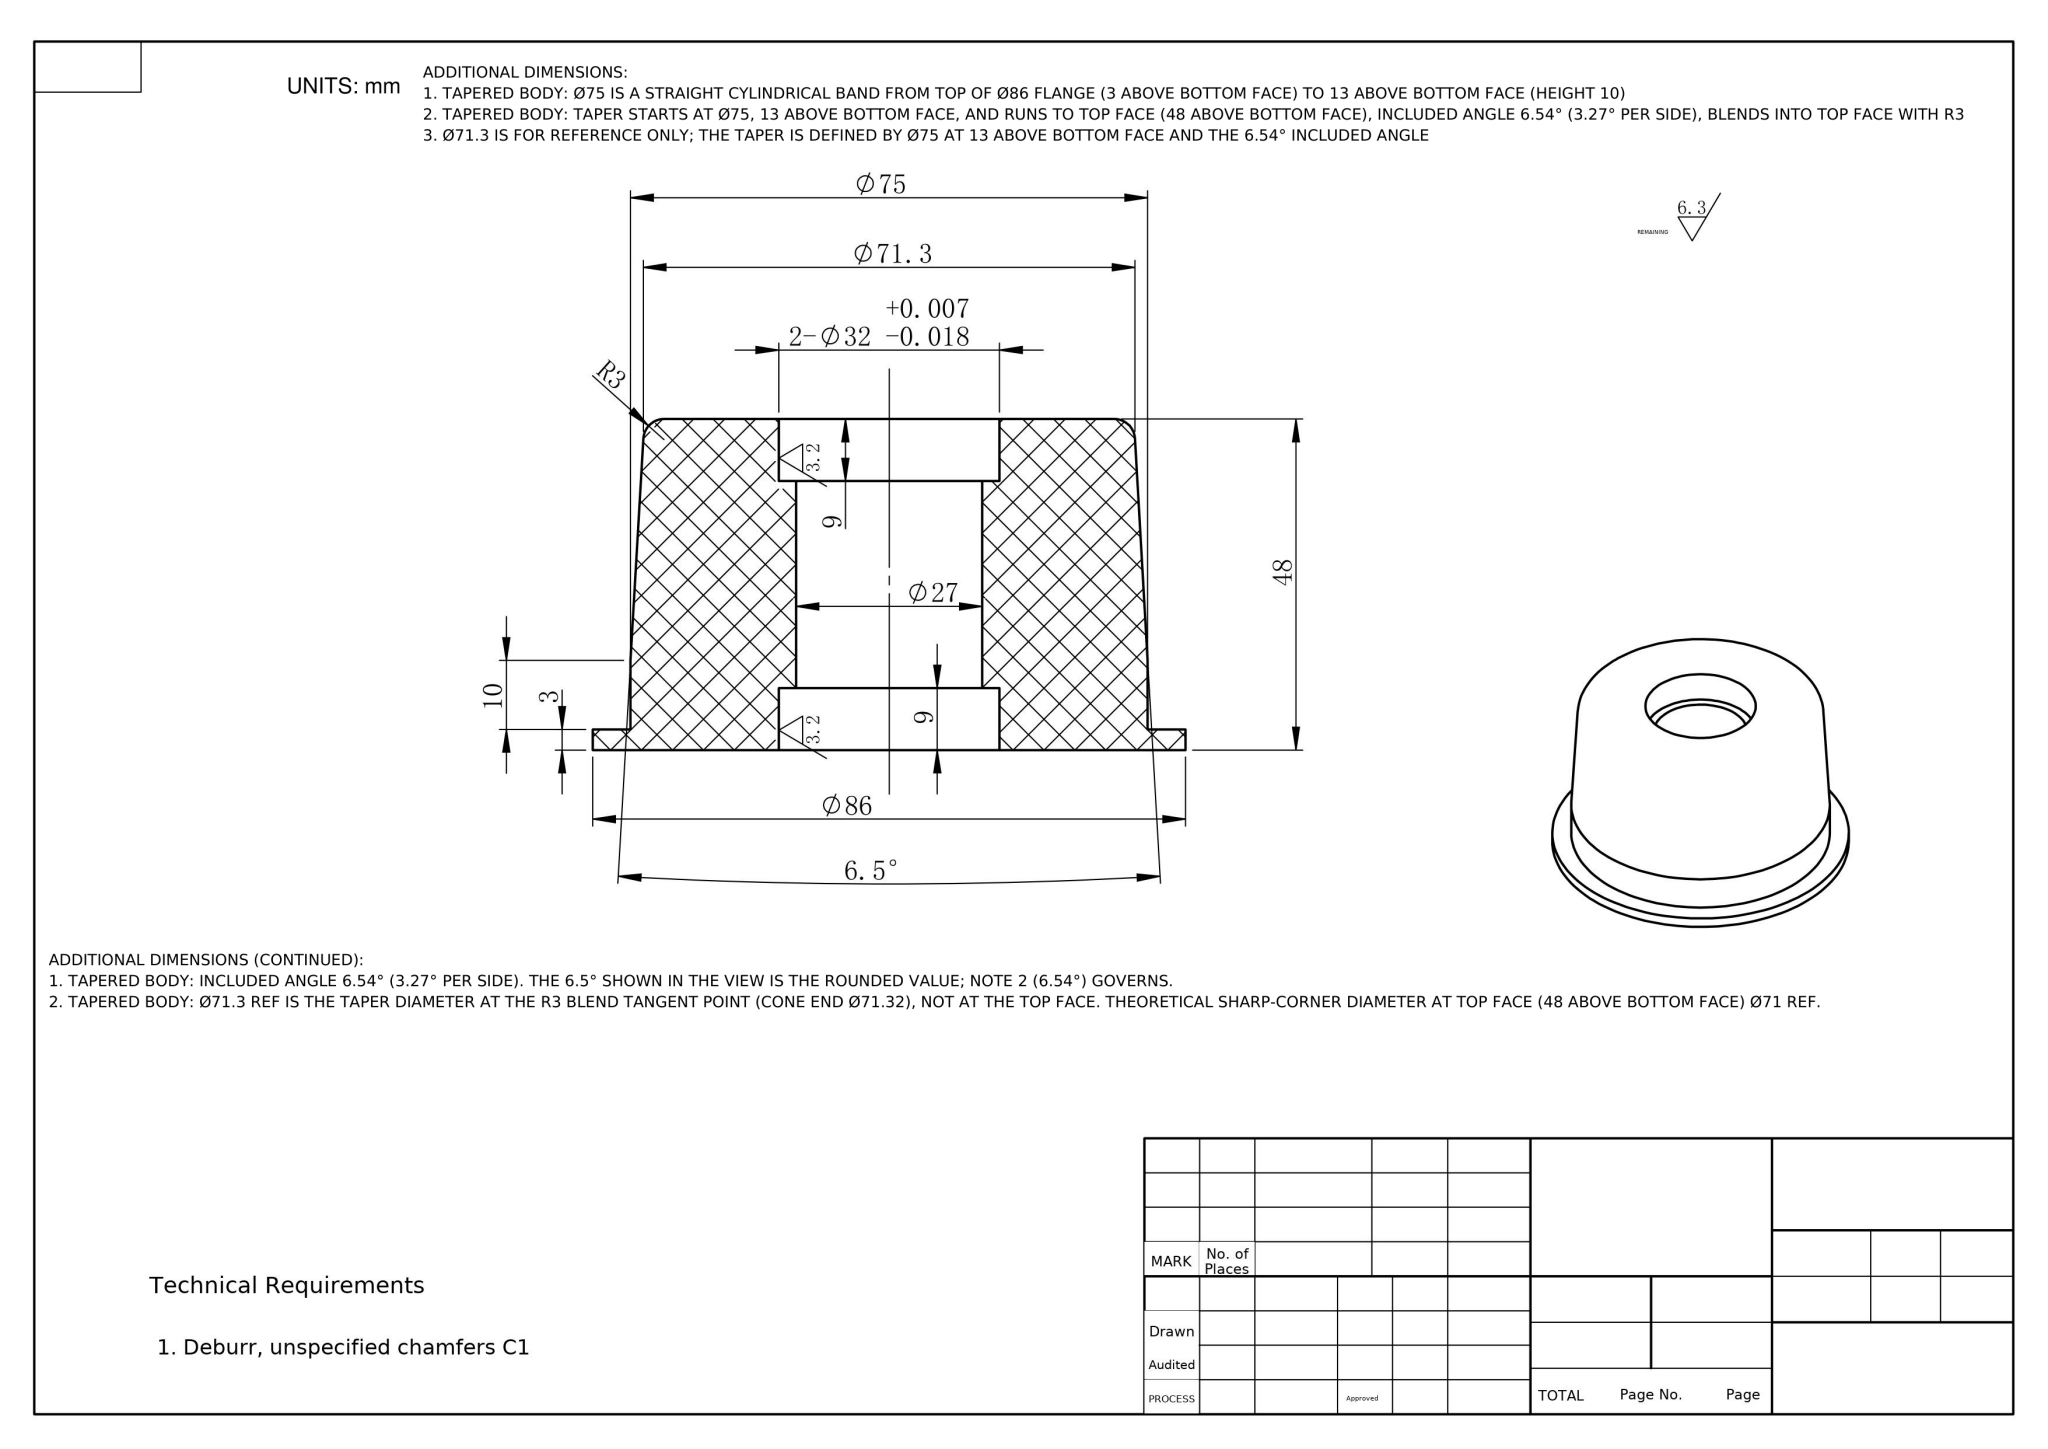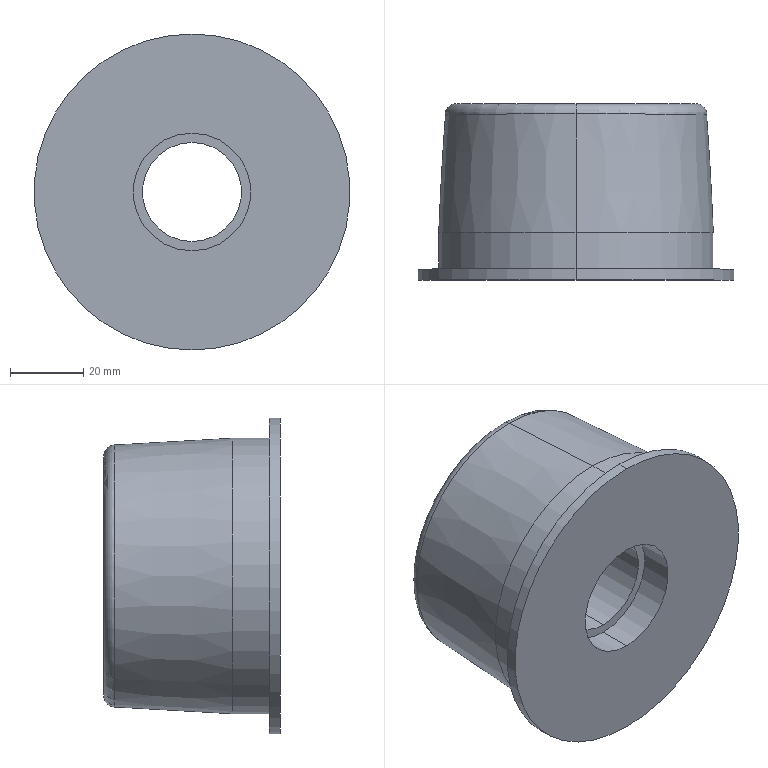Part | NX | mm | 1 solid | 19 faces | box 86 x 48 x 86 mm | volume 176107 mm3 | cylinder 10 | plane 5 | torus 2 | cone 2 | commonest cylinder face diameters 32 x4 75 x2 86 x2 27 x2
STEP:
#1=COLOUR_RGB('',0.9882,0.7373,0.5176);
#2=FILL_AREA_STYLE_COLOUR('',#1);
#3=FILL_AREA_STYLE('',(#2));
#4=SURFACE_STYLE_FILL_AREA(#3);
#5=SURFACE_SIDE_STYLE('',(#4));
#6=SURFACE_STYLE_USAGE(.BOTH.,#5);
#7=PRESENTATION_STYLE_ASSIGNMENT((#6));
#8=CARTESIAN_POINT('',(0.,13.,-37.5));
#9=VERTEX_POINT('',#8);
#10=CARTESIAN_POINT('',(0.,13.,37.5));
#11=VERTEX_POINT('',#10);
#12=CARTESIAN_POINT('',(0.,13.,0.));
#13=DIRECTION('',(0.,-1.,0.));
#14=DIRECTION('',(0.,0.,-1.));
#15=AXIS2_PLACEMENT_3D('',#12,#13,#14);
#16=CIRCLE('',#15,37.5);
#17=EDGE_CURVE('',#9,#11,#16,.T.);
#18=ORIENTED_EDGE('',*,*,#17,.T.);
#19=CARTESIAN_POINT('',(0.,3.,37.5));
#20=VERTEX_POINT('',#19);
#21=CARTESIAN_POINT('',(0.,-3.006,37.5));
#22=DIRECTION('',(0.,-1.,0.));
#23=VECTOR('',#22,1000.);
#24=LINE('',#21,#23);
#25=EDGE_CURVE('',#11,#20,#24,.T.);
#26=ORIENTED_EDGE('',*,*,#25,.T.);
#27=CARTESIAN_POINT('',(0.,3.,-37.5));
#28=VERTEX_POINT('',#27);
#29=CARTESIAN_POINT('',(0.,3.,0.));
#30=DIRECTION('',(0.,-1.,0.));
#31=DIRECTION('',(0.,0.,-1.));
#32=AXIS2_PLACEMENT_3D('',#29,#30,#31);
#33=CIRCLE('',#32,37.5);
#34=EDGE_CURVE('',#28,#20,#33,.T.);
#35=ORIENTED_EDGE('',*,*,#34,.F.);
#36=CARTESIAN_POINT('',(0.,-3.006,-37.5));
#37=DIRECTION('',(0.,-1.,0.));
#38=VECTOR('',#37,1000.);
#39=LINE('',#36,#38);
#40=EDGE_CURVE('',#9,#28,#39,.T.);
#41=ORIENTED_EDGE('',*,*,#40,.F.);
#42=EDGE_LOOP('',(#18,#26,#35,#41));
#43=FACE_OUTER_BOUND('',#42,.T.);
#44=CARTESIAN_POINT('',(0.,-3.006,0.));
#45=DIRECTION('',(0.,-1.,0.));
#46=DIRECTION('',(0.,0.,-1.));
#47=AXIS2_PLACEMENT_3D('',#44,#45,#46);
#48=CYLINDRICAL_SURFACE('',#47,37.5);
#49=ADVANCED_FACE('',(#43),#48,.T.);
#50=CARTESIAN_POINT('',(0.,3.,-43.));
#51=VERTEX_POINT('',#50);
#52=CARTESIAN_POINT('',(0.,3.,43.));
#53=VERTEX_POINT('',#52);
#54=CARTESIAN_POINT('',(0.,3.,0.));
#55=DIRECTION('',(0.,-1.,0.));
#56=DIRECTION('',(0.,0.,-1.));
#57=AXIS2_PLACEMENT_3D('',#54,#55,#56);
#58=CIRCLE('',#57,43.);
#59=EDGE_CURVE('',#51,#53,#58,.T.);
#60=ORIENTED_EDGE('',*,*,#59,.T.);
#61=CARTESIAN_POINT('',(0.,0.,43.));
#62=VERTEX_POINT('',#61);
#63=CARTESIAN_POINT('',(0.,-3.006,43.));
#64=DIRECTION('',(0.,-1.,0.));
#65=VECTOR('',#64,1000.);
#66=LINE('',#63,#65);
#67=EDGE_CURVE('',#53,#62,#66,.T.);
#68=ORIENTED_EDGE('',*,*,#67,.T.);
#69=CARTESIAN_POINT('',(0.,0.,-43.));
#70=VERTEX_POINT('',#69);
#71=CARTESIAN_POINT('',(0.,0.,0.));
#72=DIRECTION('',(0.,-1.,0.));
#73=DIRECTION('',(0.,0.,-1.));
#74=AXIS2_PLACEMENT_3D('',#71,#72,#73);
#75=CIRCLE('',#74,43.);
#76=EDGE_CURVE('',#70,#62,#75,.T.);
#77=ORIENTED_EDGE('',*,*,#76,.F.);
#78=CARTESIAN_POINT('',(0.,-3.006,-43.));
#79=DIRECTION('',(0.,-1.,0.));
#80=VECTOR('',#79,1000.);
#81=LINE('',#78,#80);
#82=EDGE_CURVE('',#51,#70,#81,.T.);
#83=ORIENTED_EDGE('',*,*,#82,.F.);
#84=EDGE_LOOP('',(#60,#68,#77,#83));
#85=FACE_OUTER_BOUND('',#84,.T.);
#86=CARTESIAN_POINT('',(0.,-3.006,0.));
#87=DIRECTION('',(0.,-1.,0.));
#88=DIRECTION('',(0.,0.,-1.));
#89=AXIS2_PLACEMENT_3D('',#86,#87,#88);
#90=CYLINDRICAL_SURFACE('',#89,43.);
#91=ADVANCED_FACE('',(#85),#90,.T.);
#92=CARTESIAN_POINT('',(0.,9.,16.));
#93=VERTEX_POINT('',#92);
#94=CARTESIAN_POINT('',(0.,9.,-16.));
#95=VERTEX_POINT('',#94);
#96=CARTESIAN_POINT('',(0.,9.,0.));
#97=DIRECTION('',(0.,-1.,0.));
#98=DIRECTION('',(0.,0.,-1.));
#99=AXIS2_PLACEMENT_3D('',#96,#97,#98);
#100=CIRCLE('',#99,16.);
#101=EDGE_CURVE('',#93,#95,#100,.T.);
#102=ORIENTED_EDGE('',*,*,#101,.F.);
#103=CARTESIAN_POINT('',(0.,0.,16.));
#104=VERTEX_POINT('',#103);
#105=CARTESIAN_POINT('',(0.,-3.006,16.));
#106=DIRECTION('',(0.,-1.,0.));
#107=VECTOR('',#106,1000.);
#108=LINE('',#105,#107);
#109=EDGE_CURVE('',#93,#104,#108,.T.);
#110=ORIENTED_EDGE('',*,*,#109,.T.);
#111=CARTESIAN_POINT('',(0.,0.,-16.));
#112=VERTEX_POINT('',#111);
#113=CARTESIAN_POINT('',(0.,0.,0.));
#114=DIRECTION('',(0.,-1.,0.));
#115=DIRECTION('',(0.,0.,-1.));
#116=AXIS2_PLACEMENT_3D('',#113,#114,#115);
#117=CIRCLE('',#116,16.);
#118=EDGE_CURVE('',#104,#112,#117,.T.);
#119=ORIENTED_EDGE('',*,*,#118,.T.);
#120=CARTESIAN_POINT('',(0.,-3.006,-16.));
#121=DIRECTION('',(0.,-1.,0.));
#122=VECTOR('',#121,1000.);
#123=LINE('',#120,#122);
#124=EDGE_CURVE('',#95,#112,#123,.T.);
#125=ORIENTED_EDGE('',*,*,#124,.F.);
#126=EDGE_LOOP('',(#102,#110,#119,#125));
#127=FACE_OUTER_BOUND('',#126,.T.);
#128=CARTESIAN_POINT('',(0.,-3.006,0.));
#129=DIRECTION('',(0.,-1.,0.));
#130=DIRECTION('',(0.,0.,-1.));
#131=AXIS2_PLACEMENT_3D('',#128,#129,#130);
#132=CYLINDRICAL_SURFACE('',#131,16.);
#133=ADVANCED_FACE('',(#127),#132,.F.);
#134=CARTESIAN_POINT('',(0.,39.,13.5));
#135=VERTEX_POINT('',#134);
#136=CARTESIAN_POINT('',(0.,39.,-13.5));
#137=VERTEX_POINT('',#136);
#138=CARTESIAN_POINT('',(0.,39.,0.));
#139=DIRECTION('',(0.,-1.,0.));
#140=DIRECTION('',(0.,0.,-1.));
#141=AXIS2_PLACEMENT_3D('',#138,#139,#140);
#142=CIRCLE('',#141,13.5);
#143=EDGE_CURVE('',#135,#137,#142,.T.);
#144=ORIENTED_EDGE('',*,*,#143,.F.);
#145=CARTESIAN_POINT('',(0.,9.,13.5));
#146=VERTEX_POINT('',#145);
#147=CARTESIAN_POINT('',(0.,-3.006,13.5));
#148=DIRECTION('',(0.,-1.,0.));
#149=VECTOR('',#148,1000.);
#150=LINE('',#147,#149);
#151=EDGE_CURVE('',#135,#146,#150,.T.);
#152=ORIENTED_EDGE('',*,*,#151,.T.);
#153=CARTESIAN_POINT('',(0.,9.,-13.5));
#154=VERTEX_POINT('',#153);
#155=CARTESIAN_POINT('',(0.,9.,0.));
#156=DIRECTION('',(0.,-1.,0.));
#157=DIRECTION('',(0.,0.,-1.));
#158=AXIS2_PLACEMENT_3D('',#155,#156,#157);
#159=CIRCLE('',#158,13.5);
#160=EDGE_CURVE('',#146,#154,#159,.T.);
#161=ORIENTED_EDGE('',*,*,#160,.T.);
#162=CARTESIAN_POINT('',(0.,-3.006,-13.5));
#163=DIRECTION('',(0.,-1.,0.));
#164=VECTOR('',#163,1000.);
#165=LINE('',#162,#164);
#166=EDGE_CURVE('',#137,#154,#165,.T.);
#167=ORIENTED_EDGE('',*,*,#166,.F.);
#168=EDGE_LOOP('',(#144,#152,#161,#167));
#169=FACE_OUTER_BOUND('',#168,.T.);
#170=CARTESIAN_POINT('',(0.,-3.006,0.));
#171=DIRECTION('',(0.,-1.,0.));
#172=DIRECTION('',(0.,0.,-1.));
#173=AXIS2_PLACEMENT_3D('',#170,#171,#172);
#174=CYLINDRICAL_SURFACE('',#173,13.5);
#175=ADVANCED_FACE('',(#169),#174,.F.);
#176=CARTESIAN_POINT('',(0.,48.,16.));
#177=VERTEX_POINT('',#176);
#178=CARTESIAN_POINT('',(0.,48.,-16.));
#179=VERTEX_POINT('',#178);
#180=CARTESIAN_POINT('',(0.,48.,0.));
#181=DIRECTION('',(0.,-1.,0.));
#182=DIRECTION('',(0.,0.,-1.));
#183=AXIS2_PLACEMENT_3D('',#180,#181,#182);
#184=CIRCLE('',#183,16.);
#185=EDGE_CURVE('',#177,#179,#184,.T.);
#186=ORIENTED_EDGE('',*,*,#185,.F.);
#187=CARTESIAN_POINT('',(0.,39.,16.));
#188=VERTEX_POINT('',#187);
#189=CARTESIAN_POINT('',(0.,-3.006,16.));
#190=DIRECTION('',(0.,-1.,0.));
#191=VECTOR('',#190,1000.);
#192=LINE('',#189,#191);
#193=EDGE_CURVE('',#177,#188,#192,.T.);
#194=ORIENTED_EDGE('',*,*,#193,.T.);
#195=CARTESIAN_POINT('',(0.,39.,-16.));
#196=VERTEX_POINT('',#195);
#197=CARTESIAN_POINT('',(0.,39.,0.));
#198=DIRECTION('',(0.,-1.,0.));
#199=DIRECTION('',(0.,0.,-1.));
#200=AXIS2_PLACEMENT_3D('',#197,#198,#199);
#201=CIRCLE('',#200,16.);
#202=EDGE_CURVE('',#188,#196,#201,.T.);
#203=ORIENTED_EDGE('',*,*,#202,.T.);
#204=CARTESIAN_POINT('',(0.,-3.006,-16.));
#205=DIRECTION('',(0.,-1.,0.));
#206=VECTOR('',#205,1000.);
#207=LINE('',#204,#206);
#208=EDGE_CURVE('',#179,#196,#207,.T.);
#209=ORIENTED_EDGE('',*,*,#208,.F.);
#210=EDGE_LOOP('',(#186,#194,#203,#209));
#211=FACE_OUTER_BOUND('',#210,.T.);
#212=CARTESIAN_POINT('',(0.,-3.006,0.));
#213=DIRECTION('',(0.,-1.,0.));
#214=DIRECTION('',(0.,0.,-1.));
#215=AXIS2_PLACEMENT_3D('',#212,#213,#214);
#216=CYLINDRICAL_SURFACE('',#215,16.);
#217=ADVANCED_FACE('',(#211),#216,.F.);
#218=CARTESIAN_POINT('',(0.,48.,-32.667));
#219=VERTEX_POINT('',#218);
#220=CARTESIAN_POINT('',(0.,48.,32.667));
#221=VERTEX_POINT('',#220);
#222=CARTESIAN_POINT('',(0.,48.,0.));
#223=DIRECTION('',(0.,-1.,0.));
#224=DIRECTION('',(0.,0.,-1.));
#225=AXIS2_PLACEMENT_3D('',#222,#223,#224);
#226=CIRCLE('',#225,32.667);
#227=EDGE_CURVE('',#219,#221,#226,.T.);
#228=ORIENTED_EDGE('',*,*,#227,.T.);
#229=CARTESIAN_POINT('',(0.,45.171,35.662));
#230=VERTEX_POINT('',#229);
#231=CARTESIAN_POINT('',(0.,45.,32.667));
#232=DIRECTION('',(1.,0.,-0.));
#233=DIRECTION('',(-0.,0.,-1.));
#234=AXIS2_PLACEMENT_3D('',#231,#232,#233);
#235=CIRCLE('',#234,3.);
#236=EDGE_CURVE('',#221,#230,#235,.T.);
#237=ORIENTED_EDGE('',*,*,#236,.T.);
#238=CARTESIAN_POINT('',(0.,45.171,-35.662));
#239=VERTEX_POINT('',#238);
#240=CARTESIAN_POINT('',(0.,45.171,0.));
#241=DIRECTION('',(0.,-1.,0.));
#242=DIRECTION('',(0.,0.,-1.));
#243=AXIS2_PLACEMENT_3D('',#240,#241,#242);
#244=CIRCLE('',#243,35.662);
#245=EDGE_CURVE('',#239,#230,#244,.T.);
#246=ORIENTED_EDGE('',*,*,#245,.F.);
#247=CARTESIAN_POINT('',(0.,45.,-32.667));
#248=DIRECTION('',(-1.,0.,0.));
#249=DIRECTION('',(0.,0.,1.));
#250=AXIS2_PLACEMENT_3D('',#247,#248,#249);
#251=CIRCLE('',#250,3.);
#252=EDGE_CURVE('',#219,#239,#251,.T.);
#253=ORIENTED_EDGE('',*,*,#252,.F.);
#254=EDGE_LOOP('',(#228,#237,#246,#253));
#255=FACE_OUTER_BOUND('',#254,.T.);
#256=CARTESIAN_POINT('',(0.,45.,0.));
#257=DIRECTION('',(0.,-1.,0.));
#258=DIRECTION('',(0.,0.,-1.));
#259=AXIS2_PLACEMENT_3D('',#256,#257,#258);
#260=TOROIDAL_SURFACE('',#259,32.667,3.);
#261=ADVANCED_FACE('',(#255),#260,.T.);
#262=ORIENTED_EDGE('',*,*,#245,.T.);
#263=CARTESIAN_POINT('',(0.,45.171,35.662));
#264=DIRECTION('',(0.,-0.9984,0.05705));
#265=VECTOR('',#264,1000.);
#266=LINE('',#263,#265);
#267=EDGE_CURVE('',#230,#11,#266,.T.);
#268=ORIENTED_EDGE('',*,*,#267,.T.);
#269=ORIENTED_EDGE('',*,*,#17,.F.);
#270=CARTESIAN_POINT('',(0.,45.171,-35.662));
#271=DIRECTION('',(0.,-0.9984,-0.05705));
#272=VECTOR('',#271,1000.);
#273=LINE('',#270,#272);
#274=EDGE_CURVE('',#239,#9,#273,.T.);
#275=ORIENTED_EDGE('',*,*,#274,.F.);
#276=EDGE_LOOP('',(#262,#268,#269,#275));
#277=FACE_OUTER_BOUND('',#276,.T.);
#278=CARTESIAN_POINT('',(0.,45.171,0.));
#279=DIRECTION('',(0.,-1.,0.));
#280=DIRECTION('',(0.,0.,-1.));
#281=AXIS2_PLACEMENT_3D('',#278,#279,#280);
#282=CONICAL_SURFACE('',#281,35.662,0.05708);
#283=ADVANCED_FACE('',(#277),#282,.T.);
#284=ORIENTED_EDGE('',*,*,#267,.F.);
#285=CARTESIAN_POINT('',(0.,45.171,0.));
#286=DIRECTION('',(0.,-1.,0.));
#287=DIRECTION('',(0.,0.,-1.));
#288=AXIS2_PLACEMENT_3D('',#285,#286,#287);
#289=CIRCLE('',#288,35.662);
#290=EDGE_CURVE('',#230,#239,#289,.T.);
#291=ORIENTED_EDGE('',*,*,#290,.T.);
#292=ORIENTED_EDGE('',*,*,#274,.T.);
#293=CARTESIAN_POINT('',(0.,13.,0.));
#294=DIRECTION('',(0.,-1.,0.));
#295=DIRECTION('',(0.,0.,-1.));
#296=AXIS2_PLACEMENT_3D('',#293,#294,#295);
#297=CIRCLE('',#296,37.5);
#298=EDGE_CURVE('',#11,#9,#297,.T.);
#299=ORIENTED_EDGE('',*,*,#298,.F.);
#300=EDGE_LOOP('',(#284,#291,#292,#299));
#301=FACE_OUTER_BOUND('',#300,.T.);
#302=CARTESIAN_POINT('',(0.,45.171,0.));
#303=DIRECTION('',(0.,-1.,0.));
#304=DIRECTION('',(0.,0.,-1.));
#305=AXIS2_PLACEMENT_3D('',#302,#303,#304);
#306=CONICAL_SURFACE('',#305,35.662,0.05708);
#307=ADVANCED_FACE('',(#301),#306,.T.);
#308=ORIENTED_EDGE('',*,*,#236,.F.);
#309=CARTESIAN_POINT('',(0.,48.,0.));
#310=DIRECTION('',(0.,-1.,0.));
#311=DIRECTION('',(0.,0.,-1.));
#312=AXIS2_PLACEMENT_3D('',#309,#310,#311);
#313=CIRCLE('',#312,32.667);
#314=EDGE_CURVE('',#221,#219,#313,.T.);
#315=ORIENTED_EDGE('',*,*,#314,.T.);
#316=ORIENTED_EDGE('',*,*,#252,.T.);
#317=ORIENTED_EDGE('',*,*,#290,.F.);
#318=EDGE_LOOP('',(#308,#315,#316,#317));
#319=FACE_OUTER_BOUND('',#318,.T.);
#320=CARTESIAN_POINT('',(0.,45.,0.));
#321=DIRECTION('',(0.,-1.,0.));
#322=DIRECTION('',(0.,0.,-1.));
#323=AXIS2_PLACEMENT_3D('',#320,#321,#322);
#324=TOROIDAL_SURFACE('',#323,32.667,3.);
#325=ADVANCED_FACE('',(#319),#324,.T.);
#326=ORIENTED_EDGE('',*,*,#227,.F.);
#327=ORIENTED_EDGE('',*,*,#314,.F.);
#328=EDGE_LOOP('',(#326,#327));
#329=FACE_OUTER_BOUND('',#328,.T.);
#330=CARTESIAN_POINT('',(0.,48.,0.));
#331=DIRECTION('',(0.,-1.,0.));
#332=DIRECTION('',(0.,0.,-1.));
#333=AXIS2_PLACEMENT_3D('',#330,#331,#332);
#334=CIRCLE('',#333,16.);
#335=EDGE_CURVE('',#179,#177,#334,.T.);
#336=ORIENTED_EDGE('',*,*,#335,.T.);
#337=ORIENTED_EDGE('',*,*,#185,.T.);
#338=EDGE_LOOP('',(#336,#337));
#339=FACE_BOUND('',#338,.T.);
#340=CARTESIAN_POINT('',(0.,48.,0.));
#341=DIRECTION('',(0.,-1.,0.));
#342=DIRECTION('',(0.,0.,-1.));
#343=AXIS2_PLACEMENT_3D('',#340,#341,#342);
#344=PLANE('',#343);
#345=ADVANCED_FACE('',(#329,#339),#344,.F.);
#346=ORIENTED_EDGE('',*,*,#193,.F.);
#347=ORIENTED_EDGE('',*,*,#335,.F.);
#348=ORIENTED_EDGE('',*,*,#208,.T.);
#349=CARTESIAN_POINT('',(0.,39.,0.));
#350=DIRECTION('',(0.,-1.,0.));
#351=DIRECTION('',(0.,0.,-1.));
#352=AXIS2_PLACEMENT_3D('',#349,#350,#351);
#353=CIRCLE('',#352,16.);
#354=EDGE_CURVE('',#196,#188,#353,.T.);
#355=ORIENTED_EDGE('',*,*,#354,.T.);
#356=EDGE_LOOP('',(#346,#347,#348,#355));
#357=FACE_OUTER_BOUND('',#356,.T.);
#358=CARTESIAN_POINT('',(0.,-3.006,0.));
#359=DIRECTION('',(0.,-1.,0.));
#360=DIRECTION('',(0.,0.,-1.));
#361=AXIS2_PLACEMENT_3D('',#358,#359,#360);
#362=CYLINDRICAL_SURFACE('',#361,16.);
#363=ADVANCED_FACE('',(#357),#362,.F.);
#364=ORIENTED_EDGE('',*,*,#354,.F.);
#365=ORIENTED_EDGE('',*,*,#202,.F.);
#366=EDGE_LOOP('',(#364,#365));
#367=FACE_OUTER_BOUND('',#366,.T.);
#368=CARTESIAN_POINT('',(0.,39.,0.));
#369=DIRECTION('',(0.,-1.,0.));
#370=DIRECTION('',(0.,0.,-1.));
#371=AXIS2_PLACEMENT_3D('',#368,#369,#370);
#372=CIRCLE('',#371,13.5);
#373=EDGE_CURVE('',#137,#135,#372,.T.);
#374=ORIENTED_EDGE('',*,*,#373,.T.);
#375=ORIENTED_EDGE('',*,*,#143,.T.);
#376=EDGE_LOOP('',(#374,#375));
#377=FACE_BOUND('',#376,.T.);
#378=CARTESIAN_POINT('',(0.,39.,0.));
#379=DIRECTION('',(0.,-1.,0.));
#380=DIRECTION('',(0.,0.,-1.));
#381=AXIS2_PLACEMENT_3D('',#378,#379,#380);
#382=PLANE('',#381);
#383=ADVANCED_FACE('',(#367,#377),#382,.F.);
#384=ORIENTED_EDGE('',*,*,#151,.F.);
#385=ORIENTED_EDGE('',*,*,#373,.F.);
#386=ORIENTED_EDGE('',*,*,#166,.T.);
#387=CARTESIAN_POINT('',(0.,9.,0.));
#388=DIRECTION('',(0.,-1.,0.));
#389=DIRECTION('',(0.,0.,-1.));
#390=AXIS2_PLACEMENT_3D('',#387,#388,#389);
#391=CIRCLE('',#390,13.5);
#392=EDGE_CURVE('',#154,#146,#391,.T.);
#393=ORIENTED_EDGE('',*,*,#392,.T.);
#394=EDGE_LOOP('',(#384,#385,#386,#393));
#395=FACE_OUTER_BOUND('',#394,.T.);
#396=CARTESIAN_POINT('',(0.,-3.006,0.));
#397=DIRECTION('',(0.,-1.,0.));
#398=DIRECTION('',(0.,0.,-1.));
#399=AXIS2_PLACEMENT_3D('',#396,#397,#398);
#400=CYLINDRICAL_SURFACE('',#399,13.5);
#401=ADVANCED_FACE('',(#395),#400,.F.);
#402=ORIENTED_EDGE('',*,*,#392,.F.);
#403=ORIENTED_EDGE('',*,*,#160,.F.);
#404=EDGE_LOOP('',(#402,#403));
#405=FACE_BOUND('',#404,.T.);
#406=CARTESIAN_POINT('',(0.,9.,0.));
#407=DIRECTION('',(0.,-1.,0.));
#408=DIRECTION('',(0.,0.,-1.));
#409=AXIS2_PLACEMENT_3D('',#406,#407,#408);
#410=CIRCLE('',#409,16.);
#411=EDGE_CURVE('',#95,#93,#410,.T.);
#412=ORIENTED_EDGE('',*,*,#411,.T.);
#413=ORIENTED_EDGE('',*,*,#101,.T.);
#414=EDGE_LOOP('',(#412,#413));
#415=FACE_OUTER_BOUND('',#414,.T.);
#416=CARTESIAN_POINT('',(0.,9.,0.));
#417=DIRECTION('',(0.,1.,0.));
#418=DIRECTION('',(0.,0.,1.));
#419=AXIS2_PLACEMENT_3D('',#416,#417,#418);
#420=PLANE('',#419);
#421=ADVANCED_FACE('',(#405,#415),#420,.F.);
#422=ORIENTED_EDGE('',*,*,#109,.F.);
#423=ORIENTED_EDGE('',*,*,#411,.F.);
#424=ORIENTED_EDGE('',*,*,#124,.T.);
#425=CARTESIAN_POINT('',(0.,0.,0.));
#426=DIRECTION('',(0.,-1.,0.));
#427=DIRECTION('',(0.,0.,-1.));
#428=AXIS2_PLACEMENT_3D('',#425,#426,#427);
#429=CIRCLE('',#428,16.);
#430=EDGE_CURVE('',#112,#104,#429,.T.);
#431=ORIENTED_EDGE('',*,*,#430,.T.);
#432=EDGE_LOOP('',(#422,#423,#424,#431));
#433=FACE_OUTER_BOUND('',#432,.T.);
#434=CARTESIAN_POINT('',(0.,-3.006,0.));
#435=DIRECTION('',(0.,-1.,0.));
#436=DIRECTION('',(0.,0.,-1.));
#437=AXIS2_PLACEMENT_3D('',#434,#435,#436);
#438=CYLINDRICAL_SURFACE('',#437,16.);
#439=ADVANCED_FACE('',(#433),#438,.F.);
#440=ORIENTED_EDGE('',*,*,#76,.T.);
#441=CARTESIAN_POINT('',(0.,0.,0.));
#442=DIRECTION('',(0.,-1.,0.));
#443=DIRECTION('',(0.,0.,-1.));
#444=AXIS2_PLACEMENT_3D('',#441,#442,#443);
#445=CIRCLE('',#444,43.);
#446=EDGE_CURVE('',#62,#70,#445,.T.);
#447=ORIENTED_EDGE('',*,*,#446,.T.);
#448=EDGE_LOOP('',(#440,#447));
#449=FACE_OUTER_BOUND('',#448,.T.);
#450=ORIENTED_EDGE('',*,*,#430,.F.);
#451=ORIENTED_EDGE('',*,*,#118,.F.);
#452=EDGE_LOOP('',(#450,#451));
#453=FACE_BOUND('',#452,.T.);
#454=CARTESIAN_POINT('',(0.,0.,0.));
#455=DIRECTION('',(0.,-1.,0.));
#456=DIRECTION('',(0.,0.,-1.));
#457=AXIS2_PLACEMENT_3D('',#454,#455,#456);
#458=PLANE('',#457);
#459=ADVANCED_FACE('',(#449,#453),#458,.T.);
#460=ORIENTED_EDGE('',*,*,#67,.F.);
#461=CARTESIAN_POINT('',(0.,3.,0.));
#462=DIRECTION('',(0.,-1.,0.));
#463=DIRECTION('',(0.,0.,-1.));
#464=AXIS2_PLACEMENT_3D('',#461,#462,#463);
#465=CIRCLE('',#464,43.);
#466=EDGE_CURVE('',#53,#51,#465,.T.);
#467=ORIENTED_EDGE('',*,*,#466,.T.);
#468=ORIENTED_EDGE('',*,*,#82,.T.);
#469=ORIENTED_EDGE('',*,*,#446,.F.);
#470=EDGE_LOOP('',(#460,#467,#468,#469));
#471=FACE_OUTER_BOUND('',#470,.T.);
#472=CARTESIAN_POINT('',(0.,-3.006,0.));
#473=DIRECTION('',(0.,-1.,0.));
#474=DIRECTION('',(0.,0.,-1.));
#475=AXIS2_PLACEMENT_3D('',#472,#473,#474);
#476=CYLINDRICAL_SURFACE('',#475,43.);
#477=ADVANCED_FACE('',(#471),#476,.T.);
#478=ORIENTED_EDGE('',*,*,#59,.F.);
#479=ORIENTED_EDGE('',*,*,#466,.F.);
#480=EDGE_LOOP('',(#478,#479));
#481=FACE_OUTER_BOUND('',#480,.T.);
#482=ORIENTED_EDGE('',*,*,#34,.T.);
#483=CARTESIAN_POINT('',(0.,3.,0.));
#484=DIRECTION('',(0.,-1.,0.));
#485=DIRECTION('',(0.,0.,-1.));
#486=AXIS2_PLACEMENT_3D('',#483,#484,#485);
#487=CIRCLE('',#486,37.5);
#488=EDGE_CURVE('',#20,#28,#487,.T.);
#489=ORIENTED_EDGE('',*,*,#488,.T.);
#490=EDGE_LOOP('',(#482,#489));
#491=FACE_BOUND('',#490,.T.);
#492=CARTESIAN_POINT('',(0.,3.,0.));
#493=DIRECTION('',(0.,-1.,0.));
#494=DIRECTION('',(0.,0.,-1.));
#495=AXIS2_PLACEMENT_3D('',#492,#493,#494);
#496=PLANE('',#495);
#497=ADVANCED_FACE('',(#481,#491),#496,.F.);
#498=ORIENTED_EDGE('',*,*,#25,.F.);
#499=ORIENTED_EDGE('',*,*,#298,.T.);
#500=ORIENTED_EDGE('',*,*,#40,.T.);
#501=ORIENTED_EDGE('',*,*,#488,.F.);
#502=EDGE_LOOP('',(#498,#499,#500,#501));
#503=FACE_OUTER_BOUND('',#502,.T.);
#504=CARTESIAN_POINT('',(0.,-3.006,0.));
#505=DIRECTION('',(0.,-1.,0.));
#506=DIRECTION('',(0.,0.,-1.));
#507=AXIS2_PLACEMENT_3D('',#504,#505,#506);
#508=CYLINDRICAL_SURFACE('',#507,37.5);
#509=ADVANCED_FACE('',(#503),#508,.T.);
#510=CLOSED_SHELL('',(#49,#91,#133,#175,#217,#261,#283,#307,#325,#345,#363,#383,#401,#421,#439,#459,#477,#497,#509));
#511=MANIFOLD_SOLID_BREP('',#510);
#512=CARTESIAN_POINT('',(0.,0.,0.));
#513=DIRECTION('',(0.,0.,1.));
#514=DIRECTION('',(1.,0.,0.));
#515=AXIS2_PLACEMENT_3D('',#512,#513,#514);
#516=(LENGTH_UNIT()NAMED_UNIT(*)SI_UNIT(.MILLI.,.METRE.));
#517=UNCERTAINTY_MEASURE_WITH_UNIT(LENGTH_MEASURE(0.00001),#516,'','');
#518=(NAMED_UNIT(*)PLANE_ANGLE_UNIT()SI_UNIT($,.RADIAN.));
#519=(NAMED_UNIT(*)SI_UNIT($,.STERADIAN.)SOLID_ANGLE_UNIT());
#520=(GEOMETRIC_REPRESENTATION_CONTEXT(3)GLOBAL_UNCERTAINTY_ASSIGNED_CONTEXT((#517))GLOBAL_UNIT_ASSIGNED_CONTEXT((#516,#518,#519))REPRESENTATION_CONTEXT('',''));
#521=ADVANCED_BREP_SHAPE_REPRESENTATION('',(#511,#515),#520);
#522=STYLED_ITEM('',(#7),#521);
#523=(LENGTH_UNIT()NAMED_UNIT(*)SI_UNIT(.MILLI.,.METRE.));
#524=UNCERTAINTY_MEASURE_WITH_UNIT(LENGTH_MEASURE(0.00001),#523,'','');
#525=(NAMED_UNIT(*)PLANE_ANGLE_UNIT()SI_UNIT($,.RADIAN.));
#526=(NAMED_UNIT(*)SI_UNIT($,.STERADIAN.)SOLID_ANGLE_UNIT());
#527=(GEOMETRIC_REPRESENTATION_CONTEXT(3)GLOBAL_UNCERTAINTY_ASSIGNED_CONTEXT((#524))GLOBAL_UNIT_ASSIGNED_CONTEXT((#523,#525,#526))REPRESENTATION_CONTEXT('',''));
#528=MECHANICAL_DESIGN_GEOMETRIC_PRESENTATION_REPRESENTATION('',(#522),#527);
#529=PRESENTATION_LAYER_ASSIGNMENT('','',(#522));
#530=COLOUR_RGB('',0.9882,0.7373,0.5176);
#531=FILL_AREA_STYLE_COLOUR('',#530);
#532=FILL_AREA_STYLE('',(#531));
#533=SURFACE_STYLE_FILL_AREA(#532);
#534=SURFACE_SIDE_STYLE('',(#533));
#535=SURFACE_STYLE_USAGE(.BOTH.,#534);
#536=PRESENTATION_STYLE_ASSIGNMENT((#535));
#537=STYLED_ITEM('',(#536),#511);
#538=(LENGTH_UNIT()NAMED_UNIT(*)SI_UNIT(.MILLI.,.METRE.));
#539=UNCERTAINTY_MEASURE_WITH_UNIT(LENGTH_MEASURE(0.00001),#538,'','');
#540=(NAMED_UNIT(*)PLANE_ANGLE_UNIT()SI_UNIT($,.RADIAN.));
#541=(NAMED_UNIT(*)SI_UNIT($,.STERADIAN.)SOLID_ANGLE_UNIT());
#542=(GEOMETRIC_REPRESENTATION_CONTEXT(3)GLOBAL_UNCERTAINTY_ASSIGNED_CONTEXT((#539))GLOBAL_UNIT_ASSIGNED_CONTEXT((#538,#540,#541))REPRESENTATION_CONTEXT('',''));
#543=MECHANICAL_DESIGN_GEOMETRIC_PRESENTATION_REPRESENTATION('',(#537),#542);
#544=PRESENTATION_LAYER_ASSIGNMENT('','',(#537));